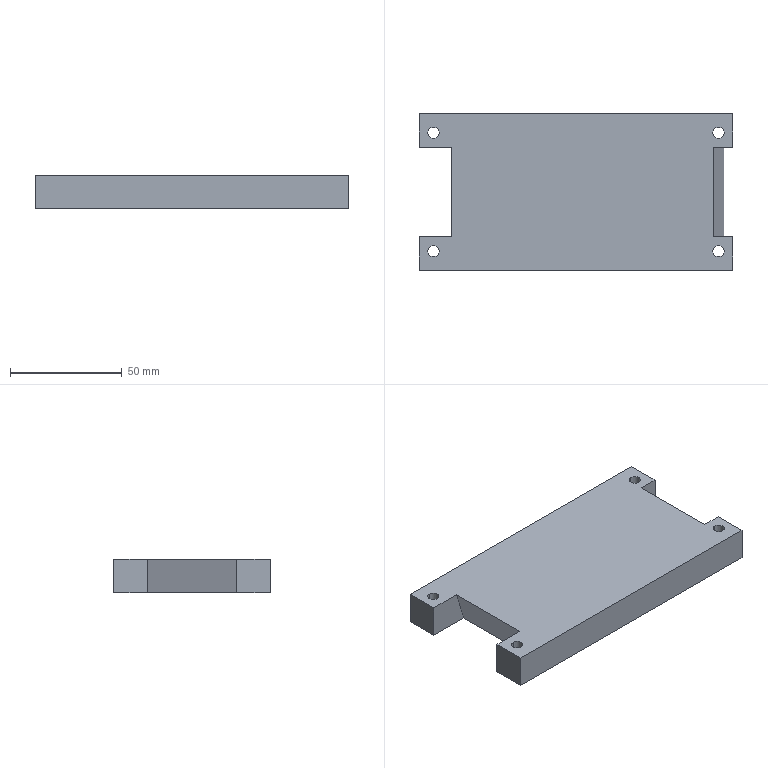Component | SolidWorks | FlatFeed-1_Part78-1 | 1 solid | 22 faces | box 140 x 70 x 15 mm | volume 132022 mm3 | plane 14 | cylinder 8 | commonest cylinder face diameters 5 x8
build123d program:
from build123d import *

# Parameters (mm, degrees)
EXTRUDE1_START        = -87.09
SKETCH5_W             = 140
SKETCH5_H             = 15
EXTRUDE1_DEPTH        = 70
EXTRUDE2_START        = -15
EXTRUDE2_DEPTH        = 40
M6_TAPPED_HOLE1_D     = 5
M6_TAPPED_HOLE1_DEPTH = 15
M6_TAPPED_HOLE1_TIP   = 1.502


with BuildPart() as part:
    # Sketch5 → Extrude1 (new body)
    with BuildSketch(Plane.XY.offset(EXTRUDE1_START)):
        with Locations((-93.422, 7930.632)):
            Rectangle(SKETCH5_W, SKETCH5_H)
    extrude(amount=-EXTRUDE1_DEPTH)

    # Sketch6 → Extrude2 (cut)
    with BuildSketch(Plane.XY.offset(-87.09).offset(EXTRUDE2_START)):
        Polygon((-163.422, 7923.132), (-159.422, 7923.132), (-149.065, 7957.007), (-185.445, 7957.007), align=None)
        Polygon((-23.422, 7923.132), (-42.422, 7923.132), (-33.086, 7953.668), (-9.562, 7951.45), align=None)
    extrude(amount=-EXTRUDE2_DEPTH, mode=Mode.SUBTRACT)

    # M6 Tapped Hole1
    with Locations(Plane(origin=(0, 7938.132, 0), x_dir=(-1, 0, 0), z_dir=(0, 1, 0))):
        with Locations((157.172, -148.59), (157.172, -95.59), (29.672, -95.59), (29.672, -148.59)):
            Hole(M6_TAPPED_HOLE1_D / 2, depth=M6_TAPPED_HOLE1_DEPTH)
            with Locations((0, 0, -(M6_TAPPED_HOLE1_DEPTH + M6_TAPPED_HOLE1_TIP / 2))):  # 118° drill point
                Cone(0, M6_TAPPED_HOLE1_D / 2, M6_TAPPED_HOLE1_TIP, mode=Mode.SUBTRACT)


solid = part.part

# Placed as in the assembly
solid = solid.moved(Location((92.879, -96.087, -7250.132), (-90, 0, 180)))
STEP:
#1=COLOUR_RGB('',0.7922,0.8196,0.9333);
#2=FILL_AREA_STYLE_COLOUR('',#1);
#3=FILL_AREA_STYLE('',(#2));
#4=SURFACE_STYLE_FILL_AREA(#3);
#5=SURFACE_SIDE_STYLE('',(#4));
#6=SURFACE_STYLE_USAGE(.BOTH.,#5);
#7=PRESENTATION_STYLE_ASSIGNMENT((#6));
#8=CARTESIAN_POINT('',(9.845,-9.731,26.496));
#9=VERTEX_POINT('',#8);
#10=CARTESIAN_POINT('',(9.845,-9.534,26.496));
#11=VERTEX_POINT('',#10);
#12=CARTESIAN_POINT('',(9.845,-9.633,26.496));
#13=DIRECTION('',(-0.,0.,1.));
#14=DIRECTION('',(0.,1.,0.));
#15=AXIS2_PLACEMENT_3D('',#12,#13,#14);
#16=CIRCLE('',#15,0.09843);
#17=EDGE_CURVE('',#9,#11,#16,.T.);
#18=ORIENTED_EDGE('',*,*,#17,.F.);
#19=CARTESIAN_POINT('',(9.845,-9.731,27.087));
#20=VERTEX_POINT('',#19);
#21=CARTESIAN_POINT('',(9.845,-9.731,27.087));
#22=DIRECTION('',(-0.,0.,1.));
#23=VECTOR('',#22,39.37);
#24=LINE('',#21,#23);
#25=EDGE_CURVE('',#9,#20,#24,.T.);
#26=ORIENTED_EDGE('',*,*,#25,.T.);
#27=CARTESIAN_POINT('',(9.845,-9.534,27.087));
#28=VERTEX_POINT('',#27);
#29=CARTESIAN_POINT('',(9.845,-9.633,27.087));
#30=DIRECTION('',(-0.,0.,1.));
#31=DIRECTION('',(0.,1.,0.));
#32=AXIS2_PLACEMENT_3D('',#29,#30,#31);
#33=CIRCLE('',#32,0.09843);
#34=EDGE_CURVE('',#20,#28,#33,.T.);
#35=ORIENTED_EDGE('',*,*,#34,.T.);
#36=CARTESIAN_POINT('',(9.845,-9.534,27.087));
#37=DIRECTION('',(-0.,0.,1.));
#38=VECTOR('',#37,39.37);
#39=LINE('',#36,#38);
#40=EDGE_CURVE('',#11,#28,#39,.T.);
#41=ORIENTED_EDGE('',*,*,#40,.F.);
#42=EDGE_LOOP('',(#18,#26,#35,#41));
#43=FACE_OUTER_BOUND('',#42,.T.);
#44=CARTESIAN_POINT('',(9.845,-9.633,27.087));
#45=DIRECTION('',(-0.,0.,1.));
#46=DIRECTION('',(0.,1.,0.));
#47=AXIS2_PLACEMENT_3D('',#44,#45,#46);
#48=CYLINDRICAL_SURFACE('',#47,0.09843);
#49=ADVANCED_FACE('',(#43),#48,.F.);
#50=CARTESIAN_POINT('',(9.845,-7.645,26.496));
#51=VERTEX_POINT('',#50);
#52=CARTESIAN_POINT('',(9.845,-7.448,26.496));
#53=VERTEX_POINT('',#52);
#54=CARTESIAN_POINT('',(9.845,-7.546,26.496));
#55=DIRECTION('',(-0.,0.,1.));
#56=DIRECTION('',(0.,1.,0.));
#57=AXIS2_PLACEMENT_3D('',#54,#55,#56);
#58=CIRCLE('',#57,0.09843);
#59=EDGE_CURVE('',#51,#53,#58,.T.);
#60=ORIENTED_EDGE('',*,*,#59,.F.);
#61=CARTESIAN_POINT('',(9.845,-7.645,27.087));
#62=VERTEX_POINT('',#61);
#63=CARTESIAN_POINT('',(9.845,-7.645,27.087));
#64=DIRECTION('',(-0.,0.,1.));
#65=VECTOR('',#64,39.37);
#66=LINE('',#63,#65);
#67=EDGE_CURVE('',#51,#62,#66,.T.);
#68=ORIENTED_EDGE('',*,*,#67,.T.);
#69=CARTESIAN_POINT('',(9.845,-7.448,27.087));
#70=VERTEX_POINT('',#69);
#71=CARTESIAN_POINT('',(9.845,-7.546,27.087));
#72=DIRECTION('',(-0.,0.,1.));
#73=DIRECTION('',(0.,1.,0.));
#74=AXIS2_PLACEMENT_3D('',#71,#72,#73);
#75=CIRCLE('',#74,0.09843);
#76=EDGE_CURVE('',#62,#70,#75,.T.);
#77=ORIENTED_EDGE('',*,*,#76,.T.);
#78=CARTESIAN_POINT('',(9.845,-7.448,27.087));
#79=DIRECTION('',(-0.,0.,1.));
#80=VECTOR('',#79,39.37);
#81=LINE('',#78,#80);
#82=EDGE_CURVE('',#53,#70,#81,.T.);
#83=ORIENTED_EDGE('',*,*,#82,.F.);
#84=EDGE_LOOP('',(#60,#68,#77,#83));
#85=FACE_OUTER_BOUND('',#84,.T.);
#86=CARTESIAN_POINT('',(9.845,-7.546,27.087));
#87=DIRECTION('',(-0.,0.,1.));
#88=DIRECTION('',(0.,1.,0.));
#89=AXIS2_PLACEMENT_3D('',#86,#87,#88);
#90=CYLINDRICAL_SURFACE('',#89,0.09843);
#91=ADVANCED_FACE('',(#85),#90,.F.);
#92=CARTESIAN_POINT('',(4.825,-7.645,26.496));
#93=VERTEX_POINT('',#92);
#94=CARTESIAN_POINT('',(4.825,-7.448,26.496));
#95=VERTEX_POINT('',#94);
#96=CARTESIAN_POINT('',(4.825,-7.546,26.496));
#97=DIRECTION('',(-0.,0.,1.));
#98=DIRECTION('',(0.,1.,0.));
#99=AXIS2_PLACEMENT_3D('',#96,#97,#98);
#100=CIRCLE('',#99,0.09843);
#101=EDGE_CURVE('',#93,#95,#100,.T.);
#102=ORIENTED_EDGE('',*,*,#101,.F.);
#103=CARTESIAN_POINT('',(4.825,-7.645,27.087));
#104=VERTEX_POINT('',#103);
#105=CARTESIAN_POINT('',(4.825,-7.645,27.087));
#106=DIRECTION('',(-0.,0.,1.));
#107=VECTOR('',#106,39.37);
#108=LINE('',#105,#107);
#109=EDGE_CURVE('',#93,#104,#108,.T.);
#110=ORIENTED_EDGE('',*,*,#109,.T.);
#111=CARTESIAN_POINT('',(4.825,-7.448,27.087));
#112=VERTEX_POINT('',#111);
#113=CARTESIAN_POINT('',(4.825,-7.546,27.087));
#114=DIRECTION('',(-0.,0.,1.));
#115=DIRECTION('',(0.,1.,0.));
#116=AXIS2_PLACEMENT_3D('',#113,#114,#115);
#117=CIRCLE('',#116,0.09843);
#118=EDGE_CURVE('',#104,#112,#117,.T.);
#119=ORIENTED_EDGE('',*,*,#118,.T.);
#120=CARTESIAN_POINT('',(4.825,-7.448,27.087));
#121=DIRECTION('',(-0.,0.,1.));
#122=VECTOR('',#121,39.37);
#123=LINE('',#120,#122);
#124=EDGE_CURVE('',#95,#112,#123,.T.);
#125=ORIENTED_EDGE('',*,*,#124,.F.);
#126=EDGE_LOOP('',(#102,#110,#119,#125));
#127=FACE_OUTER_BOUND('',#126,.T.);
#128=CARTESIAN_POINT('',(4.825,-7.546,27.087));
#129=DIRECTION('',(-0.,0.,1.));
#130=DIRECTION('',(0.,1.,0.));
#131=AXIS2_PLACEMENT_3D('',#128,#129,#130);
#132=CYLINDRICAL_SURFACE('',#131,0.09843);
#133=ADVANCED_FACE('',(#127),#132,.F.);
#134=CARTESIAN_POINT('',(4.825,-9.731,26.496));
#135=VERTEX_POINT('',#134);
#136=CARTESIAN_POINT('',(4.825,-9.534,26.496));
#137=VERTEX_POINT('',#136);
#138=CARTESIAN_POINT('',(4.825,-9.633,26.496));
#139=DIRECTION('',(-0.,0.,1.));
#140=DIRECTION('',(0.,1.,0.));
#141=AXIS2_PLACEMENT_3D('',#138,#139,#140);
#142=CIRCLE('',#141,0.09843);
#143=EDGE_CURVE('',#135,#137,#142,.T.);
#144=ORIENTED_EDGE('',*,*,#143,.F.);
#145=CARTESIAN_POINT('',(4.825,-9.731,27.087));
#146=VERTEX_POINT('',#145);
#147=CARTESIAN_POINT('',(4.825,-9.731,27.087));
#148=DIRECTION('',(-0.,0.,1.));
#149=VECTOR('',#148,39.37);
#150=LINE('',#147,#149);
#151=EDGE_CURVE('',#135,#146,#150,.T.);
#152=ORIENTED_EDGE('',*,*,#151,.T.);
#153=CARTESIAN_POINT('',(4.825,-9.534,27.087));
#154=VERTEX_POINT('',#153);
#155=CARTESIAN_POINT('',(4.825,-9.633,27.087));
#156=DIRECTION('',(-0.,0.,1.));
#157=DIRECTION('',(0.,1.,0.));
#158=AXIS2_PLACEMENT_3D('',#155,#156,#157);
#159=CIRCLE('',#158,0.09843);
#160=EDGE_CURVE('',#146,#154,#159,.T.);
#161=ORIENTED_EDGE('',*,*,#160,.T.);
#162=CARTESIAN_POINT('',(4.825,-9.534,27.087));
#163=DIRECTION('',(-0.,0.,1.));
#164=VECTOR('',#163,39.37);
#165=LINE('',#162,#164);
#166=EDGE_CURVE('',#137,#154,#165,.T.);
#167=ORIENTED_EDGE('',*,*,#166,.F.);
#168=EDGE_LOOP('',(#144,#152,#161,#167));
#169=FACE_OUTER_BOUND('',#168,.T.);
#170=CARTESIAN_POINT('',(4.825,-9.633,27.087));
#171=DIRECTION('',(-0.,0.,1.));
#172=DIRECTION('',(0.,1.,0.));
#173=AXIS2_PLACEMENT_3D('',#170,#171,#172);
#174=CYLINDRICAL_SURFACE('',#173,0.09843);
#175=ADVANCED_FACE('',(#169),#174,.F.);
#176=CARTESIAN_POINT('',(9.845,-9.633,27.087));
#177=DIRECTION('',(-0.,0.,1.));
#178=DIRECTION('',(0.,1.,0.));
#179=AXIS2_PLACEMENT_3D('',#176,#177,#178);
#180=CIRCLE('',#179,0.09843);
#181=EDGE_CURVE('',#28,#20,#180,.T.);
#182=ORIENTED_EDGE('',*,*,#181,.F.);
#183=ORIENTED_EDGE('',*,*,#34,.F.);
#184=EDGE_LOOP('',(#182,#183));
#185=FACE_BOUND('',#184,.T.);
#186=CARTESIAN_POINT('',(9.845,-7.546,27.087));
#187=DIRECTION('',(-0.,0.,1.));
#188=DIRECTION('',(0.,1.,0.));
#189=AXIS2_PLACEMENT_3D('',#186,#187,#188);
#190=CIRCLE('',#189,0.09843);
#191=EDGE_CURVE('',#70,#62,#190,.T.);
#192=ORIENTED_EDGE('',*,*,#191,.F.);
#193=ORIENTED_EDGE('',*,*,#76,.F.);
#194=EDGE_LOOP('',(#192,#193));
#195=FACE_BOUND('',#194,.T.);
#196=CARTESIAN_POINT('',(4.825,-7.546,27.087));
#197=DIRECTION('',(-0.,0.,1.));
#198=DIRECTION('',(0.,1.,0.));
#199=AXIS2_PLACEMENT_3D('',#196,#197,#198);
#200=CIRCLE('',#199,0.09843);
#201=EDGE_CURVE('',#112,#104,#200,.T.);
#202=ORIENTED_EDGE('',*,*,#201,.F.);
#203=ORIENTED_EDGE('',*,*,#118,.F.);
#204=EDGE_LOOP('',(#202,#203));
#205=FACE_BOUND('',#204,.T.);
#206=CARTESIAN_POINT('',(4.825,-9.633,27.087));
#207=DIRECTION('',(-0.,0.,1.));
#208=DIRECTION('',(0.,1.,0.));
#209=AXIS2_PLACEMENT_3D('',#206,#207,#208);
#210=CIRCLE('',#209,0.09843);
#211=EDGE_CURVE('',#154,#146,#210,.T.);
#212=ORIENTED_EDGE('',*,*,#211,.F.);
#213=ORIENTED_EDGE('',*,*,#160,.F.);
#214=EDGE_LOOP('',(#212,#213));
#215=FACE_BOUND('',#214,.T.);
#216=CARTESIAN_POINT('',(5.146,-9.377,27.087));
#217=VERTEX_POINT('',#216);
#218=CARTESIAN_POINT('',(5.146,-7.802,27.087));
#219=VERTEX_POINT('',#218);
#220=CARTESIAN_POINT('',(5.146,-9.968,27.087));
#221=DIRECTION('',(-0.,1.,-0.));
#222=VECTOR('',#221,39.37);
#223=LINE('',#220,#222);
#224=EDGE_CURVE('',#217,#219,#223,.T.);
#225=ORIENTED_EDGE('',*,*,#224,.F.);
#226=CARTESIAN_POINT('',(4.579,-9.377,27.087));
#227=VERTEX_POINT('',#226);
#228=CARTESIAN_POINT('',(10.091,-9.377,27.087));
#229=DIRECTION('',(-1.,-0.,-0.));
#230=VECTOR('',#229,39.37);
#231=LINE('',#228,#230);
#232=EDGE_CURVE('',#217,#227,#231,.T.);
#233=ORIENTED_EDGE('',*,*,#232,.T.);
#234=CARTESIAN_POINT('',(4.579,-9.968,27.087));
#235=VERTEX_POINT('',#234);
#236=CARTESIAN_POINT('',(4.579,-9.968,27.087));
#237=DIRECTION('',(-0.,1.,-0.));
#238=VECTOR('',#237,39.37);
#239=LINE('',#236,#238);
#240=EDGE_CURVE('',#235,#227,#239,.T.);
#241=ORIENTED_EDGE('',*,*,#240,.F.);
#242=CARTESIAN_POINT('',(10.091,-9.968,27.087));
#243=VERTEX_POINT('',#242);
#244=CARTESIAN_POINT('',(10.091,-9.968,27.087));
#245=DIRECTION('',(1.,0.,0.));
#246=VECTOR('',#245,39.37);
#247=LINE('',#244,#246);
#248=EDGE_CURVE('',#235,#243,#247,.T.);
#249=ORIENTED_EDGE('',*,*,#248,.T.);
#250=CARTESIAN_POINT('',(10.091,-9.377,27.087));
#251=VERTEX_POINT('',#250);
#252=CARTESIAN_POINT('',(10.091,-9.968,27.087));
#253=DIRECTION('',(-0.,1.,-0.));
#254=VECTOR('',#253,39.37);
#255=LINE('',#252,#254);
#256=EDGE_CURVE('',#243,#251,#255,.T.);
#257=ORIENTED_EDGE('',*,*,#256,.T.);
#258=CARTESIAN_POINT('',(9.753,-9.377,27.087));
#259=VERTEX_POINT('',#258);
#260=CARTESIAN_POINT('',(10.091,-9.377,27.087));
#261=DIRECTION('',(-1.,-0.,-0.));
#262=VECTOR('',#261,39.37);
#263=LINE('',#260,#262);
#264=EDGE_CURVE('',#251,#259,#263,.T.);
#265=ORIENTED_EDGE('',*,*,#264,.T.);
#266=CARTESIAN_POINT('',(9.753,-7.802,27.087));
#267=VERTEX_POINT('',#266);
#268=CARTESIAN_POINT('',(9.753,-9.968,27.087));
#269=DIRECTION('',(0.,-1.,0.));
#270=VECTOR('',#269,39.37);
#271=LINE('',#268,#270);
#272=EDGE_CURVE('',#267,#259,#271,.T.);
#273=ORIENTED_EDGE('',*,*,#272,.F.);
#274=CARTESIAN_POINT('',(10.091,-7.802,27.087));
#275=VERTEX_POINT('',#274);
#276=CARTESIAN_POINT('',(10.091,-7.802,27.087));
#277=DIRECTION('',(-1.,-0.,-0.));
#278=VECTOR('',#277,39.37);
#279=LINE('',#276,#278);
#280=EDGE_CURVE('',#275,#267,#279,.T.);
#281=ORIENTED_EDGE('',*,*,#280,.F.);
#282=CARTESIAN_POINT('',(10.091,-7.212,27.087));
#283=VERTEX_POINT('',#282);
#284=CARTESIAN_POINT('',(10.091,-9.968,27.087));
#285=DIRECTION('',(-0.,1.,-0.));
#286=VECTOR('',#285,39.37);
#287=LINE('',#284,#286);
#288=EDGE_CURVE('',#275,#283,#287,.T.);
#289=ORIENTED_EDGE('',*,*,#288,.T.);
#290=CARTESIAN_POINT('',(4.579,-7.212,27.087));
#291=VERTEX_POINT('',#290);
#292=CARTESIAN_POINT('',(10.091,-7.212,27.087));
#293=DIRECTION('',(1.,0.,0.));
#294=VECTOR('',#293,39.37);
#295=LINE('',#292,#294);
#296=EDGE_CURVE('',#291,#283,#295,.T.);
#297=ORIENTED_EDGE('',*,*,#296,.F.);
#298=CARTESIAN_POINT('',(4.579,-7.802,27.087));
#299=VERTEX_POINT('',#298);
#300=CARTESIAN_POINT('',(4.579,-9.968,27.087));
#301=DIRECTION('',(-0.,1.,-0.));
#302=VECTOR('',#301,39.37);
#303=LINE('',#300,#302);
#304=EDGE_CURVE('',#299,#291,#303,.T.);
#305=ORIENTED_EDGE('',*,*,#304,.F.);
#306=CARTESIAN_POINT('',(10.091,-7.802,27.087));
#307=DIRECTION('',(-1.,-0.,-0.));
#308=VECTOR('',#307,39.37);
#309=LINE('',#306,#308);
#310=EDGE_CURVE('',#219,#299,#309,.T.);
#311=ORIENTED_EDGE('',*,*,#310,.F.);
#312=EDGE_LOOP('',(#225,#233,#241,#249,#257,#265,#273,#281,#289,#297,#305,#311));
#313=FACE_OUTER_BOUND('',#312,.T.);
#314=CARTESIAN_POINT('',(10.091,-9.968,27.087));
#315=DIRECTION('',(-0.,0.,1.));
#316=DIRECTION('',(-0.,1.,-0.));
#317=AXIS2_PLACEMENT_3D('',#314,#315,#316);
#318=PLANE('',#317);
#319=ADVANCED_FACE('',(#185,#195,#205,#215,#313),#318,.T.);
#320=CARTESIAN_POINT('',(9.845,-9.633,26.496));
#321=DIRECTION('',(-0.,0.,1.));
#322=DIRECTION('',(0.,1.,0.));
#323=AXIS2_PLACEMENT_3D('',#320,#321,#322);
#324=CIRCLE('',#323,0.09843);
#325=EDGE_CURVE('',#11,#9,#324,.T.);
#326=ORIENTED_EDGE('',*,*,#325,.T.);
#327=ORIENTED_EDGE('',*,*,#17,.T.);
#328=EDGE_LOOP('',(#326,#327));
#329=FACE_BOUND('',#328,.T.);
#330=CARTESIAN_POINT('',(9.845,-7.546,26.496));
#331=DIRECTION('',(-0.,0.,1.));
#332=DIRECTION('',(0.,1.,0.));
#333=AXIS2_PLACEMENT_3D('',#330,#331,#332);
#334=CIRCLE('',#333,0.09843);
#335=EDGE_CURVE('',#53,#51,#334,.T.);
#336=ORIENTED_EDGE('',*,*,#335,.T.);
#337=ORIENTED_EDGE('',*,*,#59,.T.);
#338=EDGE_LOOP('',(#336,#337));
#339=FACE_BOUND('',#338,.T.);
#340=CARTESIAN_POINT('',(4.825,-7.546,26.496));
#341=DIRECTION('',(-0.,0.,1.));
#342=DIRECTION('',(0.,1.,0.));
#343=AXIS2_PLACEMENT_3D('',#340,#341,#342);
#344=CIRCLE('',#343,0.09843);
#345=EDGE_CURVE('',#95,#93,#344,.T.);
#346=ORIENTED_EDGE('',*,*,#345,.T.);
#347=ORIENTED_EDGE('',*,*,#101,.T.);
#348=EDGE_LOOP('',(#346,#347));
#349=FACE_BOUND('',#348,.T.);
#350=CARTESIAN_POINT('',(4.825,-9.633,26.496));
#351=DIRECTION('',(-0.,0.,1.));
#352=DIRECTION('',(0.,1.,0.));
#353=AXIS2_PLACEMENT_3D('',#350,#351,#352);
#354=CIRCLE('',#353,0.09843);
#355=EDGE_CURVE('',#137,#135,#354,.T.);
#356=ORIENTED_EDGE('',*,*,#355,.T.);
#357=ORIENTED_EDGE('',*,*,#143,.T.);
#358=EDGE_LOOP('',(#356,#357));
#359=FACE_BOUND('',#358,.T.);
#360=CARTESIAN_POINT('',(4.579,-9.968,26.496));
#361=VERTEX_POINT('',#360);
#362=CARTESIAN_POINT('',(4.579,-9.377,26.496));
#363=VERTEX_POINT('',#362);
#364=CARTESIAN_POINT('',(4.579,-9.968,26.496));
#365=DIRECTION('',(-0.,1.,-0.));
#366=VECTOR('',#365,39.37);
#367=LINE('',#364,#366);
#368=EDGE_CURVE('',#361,#363,#367,.T.);
#369=ORIENTED_EDGE('',*,*,#368,.T.);
#370=CARTESIAN_POINT('',(5.327,-9.377,26.496));
#371=VERTEX_POINT('',#370);
#372=CARTESIAN_POINT('',(4.579,-9.377,26.496));
#373=DIRECTION('',(-1.,-0.,-0.));
#374=VECTOR('',#373,39.37);
#375=LINE('',#372,#374);
#376=EDGE_CURVE('',#371,#363,#375,.T.);
#377=ORIENTED_EDGE('',*,*,#376,.F.);
#378=CARTESIAN_POINT('',(5.327,-7.802,26.496));
#379=VERTEX_POINT('',#378);
#380=CARTESIAN_POINT('',(5.327,-9.377,26.496));
#381=DIRECTION('',(-0.,1.,-0.));
#382=VECTOR('',#381,39.37);
#383=LINE('',#380,#382);
#384=EDGE_CURVE('',#371,#379,#383,.T.);
#385=ORIENTED_EDGE('',*,*,#384,.T.);
#386=CARTESIAN_POINT('',(4.579,-7.802,26.496));
#387=VERTEX_POINT('',#386);
#388=CARTESIAN_POINT('',(4.579,-7.802,26.496));
#389=DIRECTION('',(-1.,-0.,-0.));
#390=VECTOR('',#389,39.37);
#391=LINE('',#388,#390);
#392=EDGE_CURVE('',#379,#387,#391,.T.);
#393=ORIENTED_EDGE('',*,*,#392,.T.);
#394=CARTESIAN_POINT('',(4.579,-7.212,26.496));
#395=VERTEX_POINT('',#394);
#396=CARTESIAN_POINT('',(4.579,-9.968,26.496));
#397=DIRECTION('',(-0.,1.,-0.));
#398=VECTOR('',#397,39.37);
#399=LINE('',#396,#398);
#400=EDGE_CURVE('',#387,#395,#399,.T.);
#401=ORIENTED_EDGE('',*,*,#400,.T.);
#402=CARTESIAN_POINT('',(10.091,-7.212,26.496));
#403=VERTEX_POINT('',#402);
#404=CARTESIAN_POINT('',(10.091,-7.212,26.496));
#405=DIRECTION('',(-1.,-0.,-0.));
#406=VECTOR('',#405,39.37);
#407=LINE('',#404,#406);
#408=EDGE_CURVE('',#403,#395,#407,.T.);
#409=ORIENTED_EDGE('',*,*,#408,.F.);
#410=CARTESIAN_POINT('',(10.091,-7.802,26.496));
#411=VERTEX_POINT('',#410);
#412=CARTESIAN_POINT('',(10.091,-9.968,26.496));
#413=DIRECTION('',(-0.,1.,-0.));
#414=VECTOR('',#413,39.37);
#415=LINE('',#412,#414);
#416=EDGE_CURVE('',#411,#403,#415,.T.);
#417=ORIENTED_EDGE('',*,*,#416,.F.);
#418=CARTESIAN_POINT('',(9.933,-7.802,26.496));
#419=VERTEX_POINT('',#418);
#420=CARTESIAN_POINT('',(10.091,-7.802,26.496));
#421=DIRECTION('',(-1.,-0.,-0.));
#422=VECTOR('',#421,39.37);
#423=LINE('',#420,#422);
#424=EDGE_CURVE('',#411,#419,#423,.T.);
#425=ORIENTED_EDGE('',*,*,#424,.T.);
#426=CARTESIAN_POINT('',(9.933,-9.377,26.496));
#427=VERTEX_POINT('',#426);
#428=CARTESIAN_POINT('',(9.933,-9.377,26.496));
#429=DIRECTION('',(-0.,1.,-0.));
#430=VECTOR('',#429,39.37);
#431=LINE('',#428,#430);
#432=EDGE_CURVE('',#427,#419,#431,.T.);
#433=ORIENTED_EDGE('',*,*,#432,.F.);
#434=CARTESIAN_POINT('',(10.091,-9.377,26.496));
#435=VERTEX_POINT('',#434);
#436=CARTESIAN_POINT('',(10.091,-9.377,26.496));
#437=DIRECTION('',(-1.,-0.,-0.));
#438=VECTOR('',#437,39.37);
#439=LINE('',#436,#438);
#440=EDGE_CURVE('',#435,#427,#439,.T.);
#441=ORIENTED_EDGE('',*,*,#440,.F.);
#442=CARTESIAN_POINT('',(10.091,-9.968,26.496));
#443=VERTEX_POINT('',#442);
#444=CARTESIAN_POINT('',(10.091,-9.968,26.496));
#445=DIRECTION('',(-0.,1.,-0.));
#446=VECTOR('',#445,39.37);
#447=LINE('',#444,#446);
#448=EDGE_CURVE('',#443,#435,#447,.T.);
#449=ORIENTED_EDGE('',*,*,#448,.F.);
#450=CARTESIAN_POINT('',(10.091,-9.968,26.496));
#451=DIRECTION('',(-1.,-0.,-0.));
#452=VECTOR('',#451,39.37);
#453=LINE('',#450,#452);
#454=EDGE_CURVE('',#443,#361,#453,.T.);
#455=ORIENTED_EDGE('',*,*,#454,.T.);
#456=EDGE_LOOP('',(#369,#377,#385,#393,#401,#409,#417,#425,#433,#441,#449,#455));
#457=FACE_OUTER_BOUND('',#456,.T.);
#458=CARTESIAN_POINT('',(10.091,-9.968,26.496));
#459=DIRECTION('',(0.,-0.,-1.));
#460=DIRECTION('',(0.,-1.,0.));
#461=AXIS2_PLACEMENT_3D('',#458,#459,#460);
#462=PLANE('',#461);
#463=ADVANCED_FACE('',(#329,#339,#349,#359,#457),#462,.T.);
#464=ORIENTED_EDGE('',*,*,#240,.T.);
#465=CARTESIAN_POINT('',(4.579,-9.377,27.087));
#466=DIRECTION('',(0.,-0.,-1.));
#467=VECTOR('',#466,39.37);
#468=LINE('',#465,#467);
#469=EDGE_CURVE('',#227,#363,#468,.T.);
#470=ORIENTED_EDGE('',*,*,#469,.T.);
#471=ORIENTED_EDGE('',*,*,#368,.F.);
#472=CARTESIAN_POINT('',(4.579,-9.968,27.087));
#473=DIRECTION('',(-0.,0.,1.));
#474=VECTOR('',#473,39.37);
#475=LINE('',#472,#474);
#476=EDGE_CURVE('',#361,#235,#475,.T.);
#477=ORIENTED_EDGE('',*,*,#476,.T.);
#478=EDGE_LOOP('',(#464,#470,#471,#477));
#479=FACE_OUTER_BOUND('',#478,.T.);
#480=CARTESIAN_POINT('',(4.579,-9.968,27.087));
#481=DIRECTION('',(-1.,-0.,-0.));
#482=DIRECTION('',(0.,-1.,0.));
#483=AXIS2_PLACEMENT_3D('',#480,#481,#482);
#484=PLANE('',#483);
#485=ADVANCED_FACE('',(#479),#484,.T.);
#486=ORIENTED_EDGE('',*,*,#448,.T.);
#487=CARTESIAN_POINT('',(10.091,-9.377,27.087));
#488=DIRECTION('',(-0.,0.,1.));
#489=VECTOR('',#488,39.37);
#490=LINE('',#487,#489);
#491=EDGE_CURVE('',#435,#251,#490,.T.);
#492=ORIENTED_EDGE('',*,*,#491,.T.);
#493=ORIENTED_EDGE('',*,*,#256,.F.);
#494=CARTESIAN_POINT('',(10.091,-9.968,27.087));
#495=DIRECTION('',(0.,-0.,-1.));
#496=VECTOR('',#495,39.37);
#497=LINE('',#494,#496);
#498=EDGE_CURVE('',#243,#443,#497,.T.);
#499=ORIENTED_EDGE('',*,*,#498,.T.);
#500=EDGE_LOOP('',(#486,#492,#493,#499));
#501=FACE_OUTER_BOUND('',#500,.T.);
#502=CARTESIAN_POINT('',(10.091,-9.968,27.087));
#503=DIRECTION('',(1.,0.,0.));
#504=DIRECTION('',(-0.,1.,-0.));
#505=AXIS2_PLACEMENT_3D('',#502,#503,#504);
#506=PLANE('',#505);
#507=ADVANCED_FACE('',(#501),#506,.T.);
#508=CARTESIAN_POINT('',(10.091,-7.802,27.087));
#509=DIRECTION('',(-0.,0.,1.));
#510=VECTOR('',#509,39.37);
#511=LINE('',#508,#510);
#512=EDGE_CURVE('',#411,#275,#511,.T.);
#513=ORIENTED_EDGE('',*,*,#512,.F.);
#514=ORIENTED_EDGE('',*,*,#416,.T.);
#515=CARTESIAN_POINT('',(10.091,-7.212,27.087));
#516=DIRECTION('',(0.,-0.,-1.));
#517=VECTOR('',#516,39.37);
#518=LINE('',#515,#517);
#519=EDGE_CURVE('',#283,#403,#518,.T.);
#520=ORIENTED_EDGE('',*,*,#519,.F.);
#521=ORIENTED_EDGE('',*,*,#288,.F.);
#522=EDGE_LOOP('',(#513,#514,#520,#521));
#523=FACE_OUTER_BOUND('',#522,.T.);
#524=CARTESIAN_POINT('',(10.091,-9.968,27.087));
#525=DIRECTION('',(1.,0.,0.));
#526=DIRECTION('',(-0.,1.,-0.));
#527=AXIS2_PLACEMENT_3D('',#524,#525,#526);
#528=PLANE('',#527);
#529=ADVANCED_FACE('',(#523),#528,.T.);
#530=CARTESIAN_POINT('',(4.579,-7.802,27.087));
#531=DIRECTION('',(0.,-0.,-1.));
#532=VECTOR('',#531,39.37);
#533=LINE('',#530,#532);
#534=EDGE_CURVE('',#299,#387,#533,.T.);
#535=ORIENTED_EDGE('',*,*,#534,.F.);
#536=ORIENTED_EDGE('',*,*,#304,.T.);
#537=CARTESIAN_POINT('',(4.579,-7.212,27.087));
#538=DIRECTION('',(-0.,0.,1.));
#539=VECTOR('',#538,39.37);
#540=LINE('',#537,#539);
#541=EDGE_CURVE('',#395,#291,#540,.T.);
#542=ORIENTED_EDGE('',*,*,#541,.F.);
#543=ORIENTED_EDGE('',*,*,#400,.F.);
#544=EDGE_LOOP('',(#535,#536,#542,#543));
#545=FACE_OUTER_BOUND('',#544,.T.);
#546=CARTESIAN_POINT('',(4.579,-9.968,27.087));
#547=DIRECTION('',(-1.,-0.,-0.));
#548=DIRECTION('',(0.,-1.,0.));
#549=AXIS2_PLACEMENT_3D('',#546,#547,#548);
#550=PLANE('',#549);
#551=ADVANCED_FACE('',(#545),#550,.T.);
#552=ORIENTED_EDGE('',*,*,#498,.F.);
#553=ORIENTED_EDGE('',*,*,#248,.F.);
#554=ORIENTED_EDGE('',*,*,#476,.F.);
#555=ORIENTED_EDGE('',*,*,#454,.F.);
#556=EDGE_LOOP('',(#552,#553,#554,#555));
#557=FACE_OUTER_BOUND('',#556,.T.);
#558=CARTESIAN_POINT('',(10.091,-9.968,26.496));
#559=DIRECTION('',(-0.,1.,-0.));
#560=DIRECTION('',(-1.,-0.,-0.));
#561=AXIS2_PLACEMENT_3D('',#558,#559,#560);
#562=PLANE('',#561);
#563=ADVANCED_FACE('',(#557),#562,.F.);
#564=ORIENTED_EDGE('',*,*,#519,.T.);
#565=ORIENTED_EDGE('',*,*,#408,.T.);
#566=ORIENTED_EDGE('',*,*,#541,.T.);
#567=ORIENTED_EDGE('',*,*,#296,.T.);
#568=EDGE_LOOP('',(#564,#565,#566,#567));
#569=FACE_OUTER_BOUND('',#568,.T.);
#570=CARTESIAN_POINT('',(10.091,-7.212,26.496));
#571=DIRECTION('',(-0.,1.,-0.));
#572=DIRECTION('',(-1.,-0.,-0.));
#573=AXIS2_PLACEMENT_3D('',#570,#571,#572);
#574=PLANE('',#573);
#575=ADVANCED_FACE('',(#569),#574,.T.);
#576=ORIENTED_EDGE('',*,*,#272,.T.);
#577=CARTESIAN_POINT('',(9.933,-9.377,26.496));
#578=DIRECTION('',(-0.2924,0.,0.9563));
#579=VECTOR('',#578,39.37);
#580=LINE('',#577,#579);
#581=EDGE_CURVE('',#427,#259,#580,.T.);
#582=ORIENTED_EDGE('',*,*,#581,.F.);
#583=ORIENTED_EDGE('',*,*,#432,.T.);
#584=CARTESIAN_POINT('',(9.933,-7.802,26.496));
#585=DIRECTION('',(-0.2924,0.,0.9563));
#586=VECTOR('',#585,39.37);
#587=LINE('',#584,#586);
#588=EDGE_CURVE('',#419,#267,#587,.T.);
#589=ORIENTED_EDGE('',*,*,#588,.T.);
#590=EDGE_LOOP('',(#576,#582,#583,#589));
#591=FACE_OUTER_BOUND('',#590,.T.);
#592=CARTESIAN_POINT('',(9.933,-9.377,26.496));
#593=DIRECTION('',(-0.9563,-0.,-0.2924));
#594=DIRECTION('',(-0.2924,0.,0.9563));
#595=AXIS2_PLACEMENT_3D('',#592,#593,#594);
#596=PLANE('',#595);
#597=ADVANCED_FACE('',(#591),#596,.F.);
#598=ORIENTED_EDGE('',*,*,#440,.T.);
#599=ORIENTED_EDGE('',*,*,#581,.T.);
#600=ORIENTED_EDGE('',*,*,#264,.F.);
#601=ORIENTED_EDGE('',*,*,#491,.F.);
#602=EDGE_LOOP('',(#598,#599,#600,#601));
#603=FACE_OUTER_BOUND('',#602,.T.);
#604=CARTESIAN_POINT('',(10.091,-9.377,26.496));
#605=DIRECTION('',(-0.,1.,-0.));
#606=DIRECTION('',(-1.,-0.,-0.));
#607=AXIS2_PLACEMENT_3D('',#604,#605,#606);
#608=PLANE('',#607);
#609=ADVANCED_FACE('',(#603),#608,.T.);
#610=ORIENTED_EDGE('',*,*,#512,.T.);
#611=ORIENTED_EDGE('',*,*,#280,.T.);
#612=ORIENTED_EDGE('',*,*,#588,.F.);
#613=ORIENTED_EDGE('',*,*,#424,.F.);
#614=EDGE_LOOP('',(#610,#611,#612,#613));
#615=FACE_OUTER_BOUND('',#614,.T.);
#616=CARTESIAN_POINT('',(10.091,-7.802,26.496));
#617=DIRECTION('',(-0.,1.,-0.));
#618=DIRECTION('',(-1.,-0.,-0.));
#619=AXIS2_PLACEMENT_3D('',#616,#617,#618);
#620=PLANE('',#619);
#621=ADVANCED_FACE('',(#615),#620,.F.);
#622=ORIENTED_EDGE('',*,*,#224,.T.);
#623=CARTESIAN_POINT('',(5.327,-7.802,26.496));
#624=DIRECTION('',(0.2924,-0.,-0.9563));
#625=VECTOR('',#624,39.37);
#626=LINE('',#623,#625);
#627=EDGE_CURVE('',#219,#379,#626,.T.);
#628=ORIENTED_EDGE('',*,*,#627,.T.);
#629=ORIENTED_EDGE('',*,*,#384,.F.);
#630=CARTESIAN_POINT('',(5.327,-9.377,26.496));
#631=DIRECTION('',(0.2924,-0.,-0.9563));
#632=VECTOR('',#631,39.37);
#633=LINE('',#630,#632);
#634=EDGE_CURVE('',#217,#371,#633,.T.);
#635=ORIENTED_EDGE('',*,*,#634,.F.);
#636=EDGE_LOOP('',(#622,#628,#629,#635));
#637=FACE_OUTER_BOUND('',#636,.T.);
#638=CARTESIAN_POINT('',(5.327,-9.377,26.496));
#639=DIRECTION('',(0.9563,0.,0.2924));
#640=DIRECTION('',(0.2924,-0.,-0.9563));
#641=AXIS2_PLACEMENT_3D('',#638,#639,#640);
#642=PLANE('',#641);
#643=ADVANCED_FACE('',(#637),#642,.F.);
#644=ORIENTED_EDGE('',*,*,#634,.T.);
#645=ORIENTED_EDGE('',*,*,#376,.T.);
#646=ORIENTED_EDGE('',*,*,#469,.F.);
#647=ORIENTED_EDGE('',*,*,#232,.F.);
#648=EDGE_LOOP('',(#644,#645,#646,#647));
#649=FACE_OUTER_BOUND('',#648,.T.);
#650=CARTESIAN_POINT('',(4.033,-9.377,27.611));
#651=DIRECTION('',(-0.,1.,-0.));
#652=DIRECTION('',(-1.,-0.,-0.));
#653=AXIS2_PLACEMENT_3D('',#650,#651,#652);
#654=PLANE('',#653);
#655=ADVANCED_FACE('',(#649),#654,.T.);
#656=ORIENTED_EDGE('',*,*,#310,.T.);
#657=ORIENTED_EDGE('',*,*,#534,.T.);
#658=ORIENTED_EDGE('',*,*,#392,.F.);
#659=ORIENTED_EDGE('',*,*,#627,.F.);
#660=EDGE_LOOP('',(#656,#657,#658,#659));
#661=FACE_OUTER_BOUND('',#660,.T.);
#662=CARTESIAN_POINT('',(4.033,-7.802,27.611));
#663=DIRECTION('',(-0.,1.,-0.));
#664=DIRECTION('',(-1.,-0.,-0.));
#665=AXIS2_PLACEMENT_3D('',#662,#663,#664);
#666=PLANE('',#665);
#667=ADVANCED_FACE('',(#661),#666,.F.);
#668=ORIENTED_EDGE('',*,*,#151,.F.);
#669=ORIENTED_EDGE('',*,*,#355,.F.);
#670=ORIENTED_EDGE('',*,*,#166,.T.);
#671=ORIENTED_EDGE('',*,*,#211,.T.);
#672=EDGE_LOOP('',(#668,#669,#670,#671));
#673=FACE_OUTER_BOUND('',#672,.T.);
#674=CARTESIAN_POINT('',(4.825,-9.633,27.087));
#675=DIRECTION('',(-0.,0.,1.));
#676=DIRECTION('',(0.,1.,0.));
#677=AXIS2_PLACEMENT_3D('',#674,#675,#676);
#678=CYLINDRICAL_SURFACE('',#677,0.09843);
#679=ADVANCED_FACE('',(#673),#678,.F.);
#680=ORIENTED_EDGE('',*,*,#109,.F.);
#681=ORIENTED_EDGE('',*,*,#345,.F.);
#682=ORIENTED_EDGE('',*,*,#124,.T.);
#683=ORIENTED_EDGE('',*,*,#201,.T.);
#684=EDGE_LOOP('',(#680,#681,#682,#683));
#685=FACE_OUTER_BOUND('',#684,.T.);
#686=CARTESIAN_POINT('',(4.825,-7.546,27.087));
#687=DIRECTION('',(-0.,0.,1.));
#688=DIRECTION('',(0.,1.,0.));
#689=AXIS2_PLACEMENT_3D('',#686,#687,#688);
#690=CYLINDRICAL_SURFACE('',#689,0.09843);
#691=ADVANCED_FACE('',(#685),#690,.F.);
#692=ORIENTED_EDGE('',*,*,#67,.F.);
#693=ORIENTED_EDGE('',*,*,#335,.F.);
#694=ORIENTED_EDGE('',*,*,#82,.T.);
#695=ORIENTED_EDGE('',*,*,#191,.T.);
#696=EDGE_LOOP('',(#692,#693,#694,#695));
#697=FACE_OUTER_BOUND('',#696,.T.);
#698=CARTESIAN_POINT('',(9.845,-7.546,27.087));
#699=DIRECTION('',(-0.,0.,1.));
#700=DIRECTION('',(0.,1.,0.));
#701=AXIS2_PLACEMENT_3D('',#698,#699,#700);
#702=CYLINDRICAL_SURFACE('',#701,0.09843);
#703=ADVANCED_FACE('',(#697),#702,.F.);
#704=ORIENTED_EDGE('',*,*,#25,.F.);
#705=ORIENTED_EDGE('',*,*,#325,.F.);
#706=ORIENTED_EDGE('',*,*,#40,.T.);
#707=ORIENTED_EDGE('',*,*,#181,.T.);
#708=EDGE_LOOP('',(#704,#705,#706,#707));
#709=FACE_OUTER_BOUND('',#708,.T.);
#710=CARTESIAN_POINT('',(9.845,-9.633,27.087));
#711=DIRECTION('',(-0.,0.,1.));
#712=DIRECTION('',(0.,1.,0.));
#713=AXIS2_PLACEMENT_3D('',#710,#711,#712);
#714=CYLINDRICAL_SURFACE('',#713,0.09843);
#715=ADVANCED_FACE('',(#709),#714,.F.);
#716=CLOSED_SHELL('',(#49,#91,#133,#175,#319,#463,#485,#507,#529,#551,#563,#575,#597,#609,#621,#643,#655,#667,#679,#691,#703,#715));
#717=MANIFOLD_SOLID_BREP('',#716);
#718=STYLED_ITEM('',(#7),#717);
#719=PRESENTATION_LAYER_ASSIGNMENT('','',(#718));
#720=(LENGTH_UNIT()NAMED_UNIT(*)SI_UNIT($,.METRE.));
#721=LENGTH_MEASURE_WITH_UNIT(LENGTH_MEASURE(0.0254),#720);
#722=DIMENSIONAL_EXPONENTS(1.,0.,0.,0.,0.,0.,0.);
#723=(CONVERSION_BASED_UNIT('',#721)LENGTH_UNIT()NAMED_UNIT(#722));
#724=UNCERTAINTY_MEASURE_WITH_UNIT(LENGTH_MEASURE(0.00001),#723,'','');
#725=(NAMED_UNIT(*)PLANE_ANGLE_UNIT()SI_UNIT($,.RADIAN.));
#726=(NAMED_UNIT(*)SI_UNIT($,.STERADIAN.)SOLID_ANGLE_UNIT());
#727=(GEOMETRIC_REPRESENTATION_CONTEXT(3)GLOBAL_UNCERTAINTY_ASSIGNED_CONTEXT((#724))GLOBAL_UNIT_ASSIGNED_CONTEXT((#723,#725,#726))REPRESENTATION_CONTEXT('',''));
#728=MECHANICAL_DESIGN_GEOMETRIC_PRESENTATION_REPRESENTATION('',(#718),#727);
#729=CARTESIAN_POINT('',(0.,0.,0.));
#730=DIRECTION('',(0.,0.,1.));
#731=DIRECTION('',(1.,0.,0.));
#732=AXIS2_PLACEMENT_3D('',#729,#730,#731);
#733=(LENGTH_UNIT()NAMED_UNIT(*)SI_UNIT($,.METRE.));
#734=LENGTH_MEASURE_WITH_UNIT(LENGTH_MEASURE(0.0254),#733);
#735=DIMENSIONAL_EXPONENTS(1.,0.,0.,0.,0.,0.,0.);
#736=(CONVERSION_BASED_UNIT('',#734)LENGTH_UNIT()NAMED_UNIT(#735));
#737=UNCERTAINTY_MEASURE_WITH_UNIT(LENGTH_MEASURE(0.00001),#736,'','');
#738=(NAMED_UNIT(*)PLANE_ANGLE_UNIT()SI_UNIT($,.RADIAN.));
#739=(NAMED_UNIT(*)SI_UNIT($,.STERADIAN.)SOLID_ANGLE_UNIT());
#740=(GEOMETRIC_REPRESENTATION_CONTEXT(3)GLOBAL_UNCERTAINTY_ASSIGNED_CONTEXT((#737))GLOBAL_UNIT_ASSIGNED_CONTEXT((#736,#738,#739))REPRESENTATION_CONTEXT('',''));
#741=ADVANCED_BREP_SHAPE_REPRESENTATION('',(#717,#732),#740);